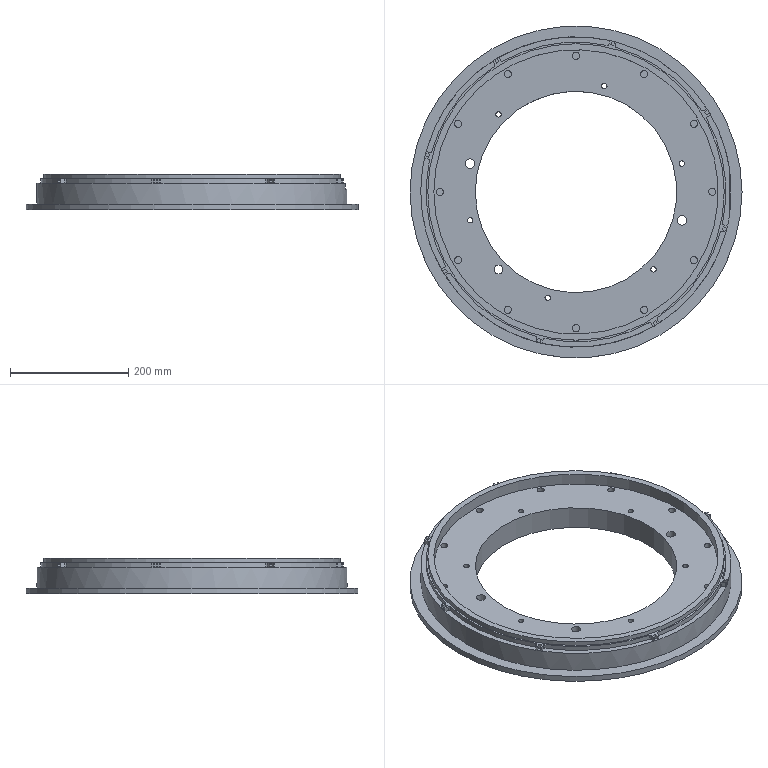CAM job | NX | mm | 3-axis | 1 set-up | 8 operations | part box 560.53 x 560.53 x 60.57
set-up 1
1. Cavity Milling | Mill Mill5 D4 | CAVITY_MILL_1 | path 224.875 mm | 2.142 min
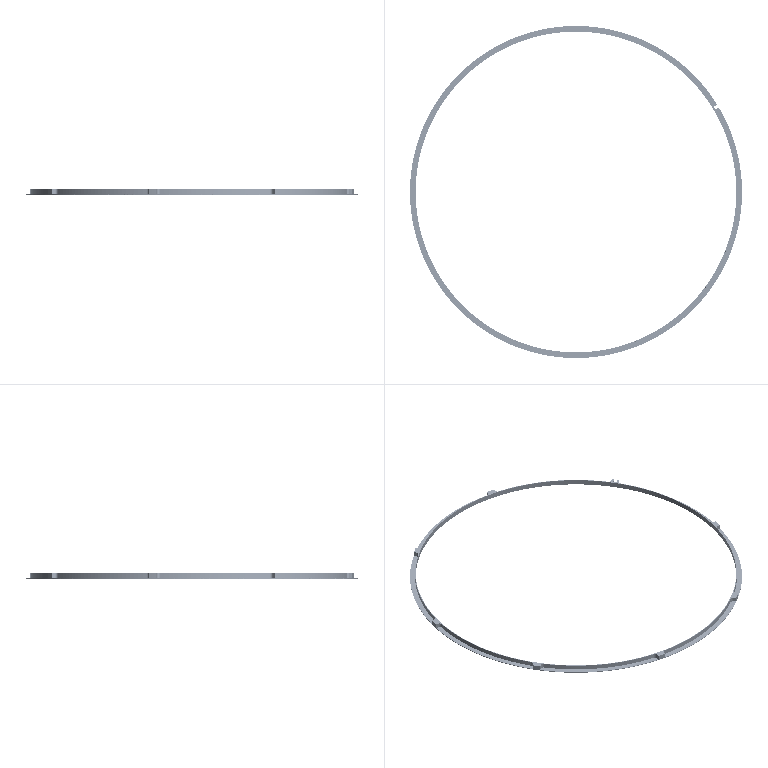2. Cavity Milling | Mill Mill5 D4 | CAVITY_MILL_1_COPY | path 224.875 mm | 2.142 min
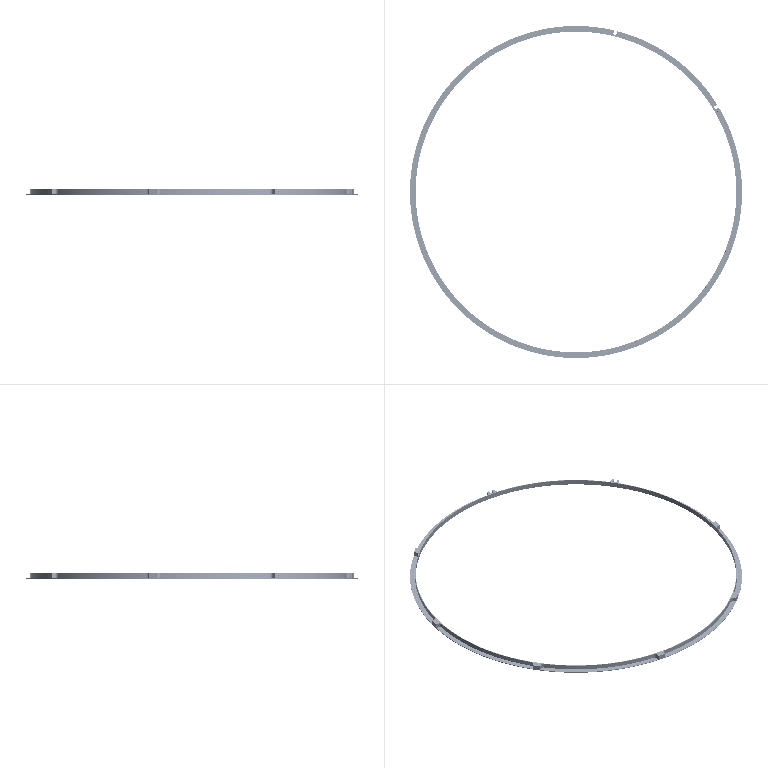3. Cavity Milling | Mill Mill5 D4 | CAVITY_MILL_1_COPY_1 | path 224.875 mm | 2.142 min
4. Cavity Milling | Mill Mill5 D4 | CAVITY_MILL_1_COPY_2 | path 224.875 mm | 2.142 min
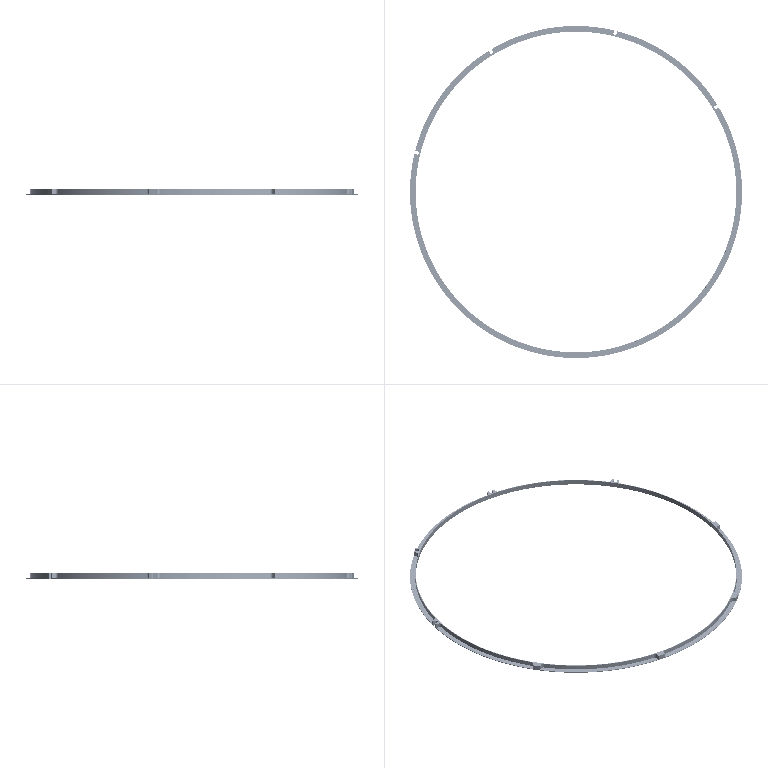5. Cavity Milling | Mill Mill5 D4 | CAVITY_MILL_1_COPY_3 | path 224.875 mm | 2.142 min
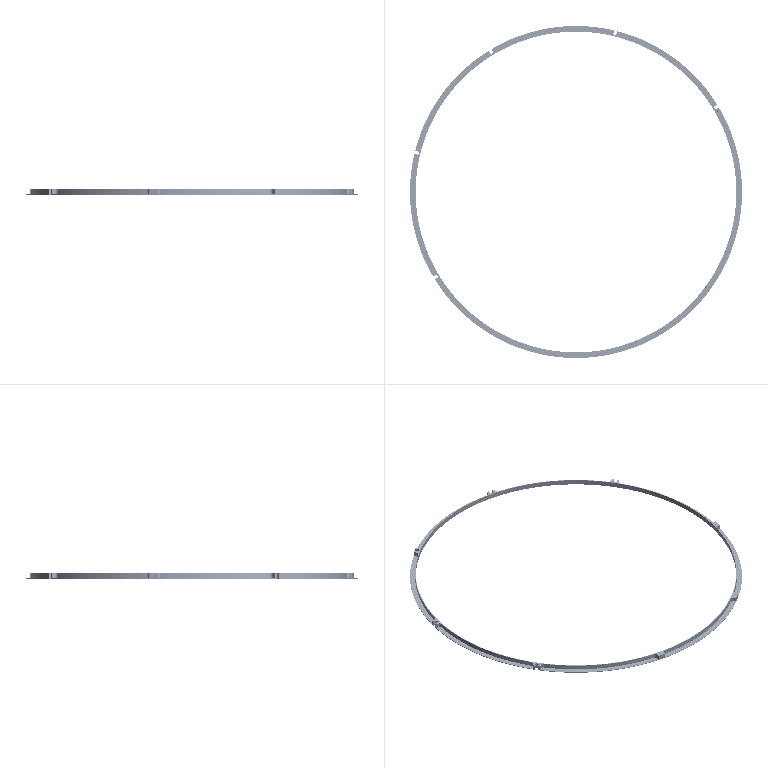6. Cavity Milling | Mill Mill5 D4 | CAVITY_MILL_1_COPY_4 | path 224.875 mm | 2.142 min
7. Cavity Milling | Mill Mill5 D4 | CAVITY_MILL_1_COPY_5 | path 224.875 mm | 2.142 min
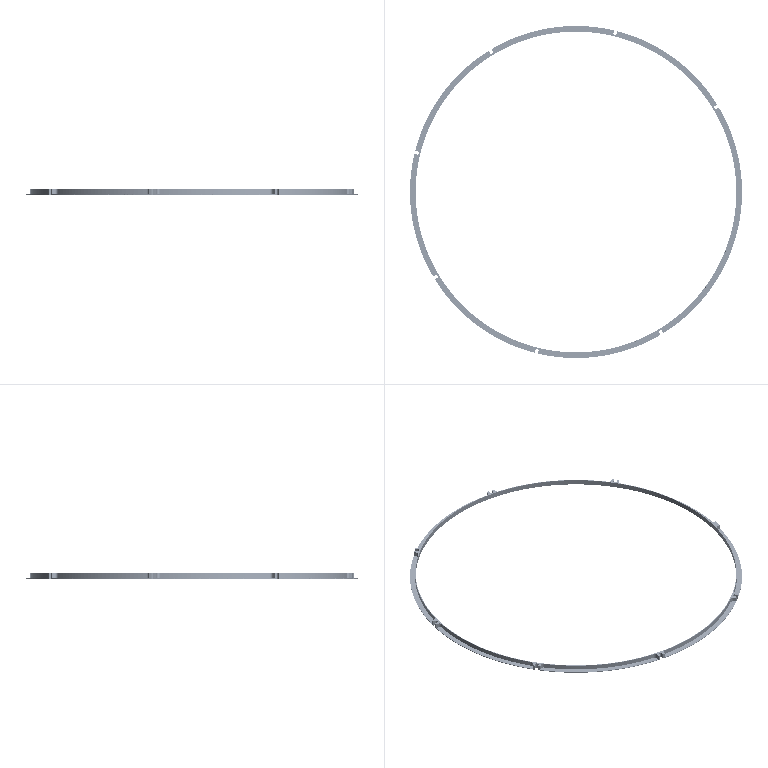8. Cavity Milling | Mill Mill5 D4 | CAVITY_MILL_1_COPY_6 | path 224.875 mm | 2.142 min